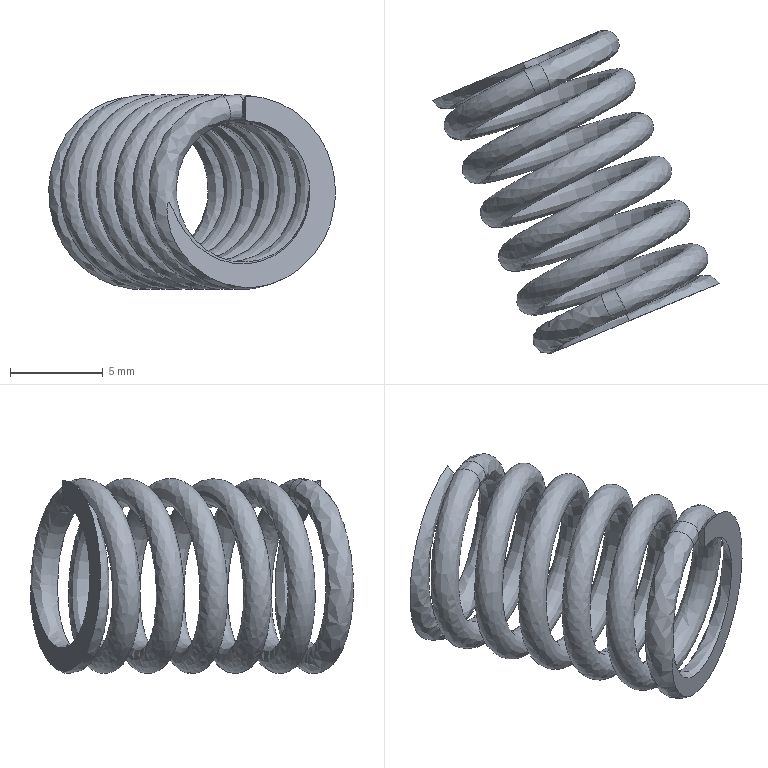Component | NX | SPRING_CYLINDER_COMPRESSION_1 | 1 solid | 9 faces | volume 321 mm3 | spline 5 | plane 4